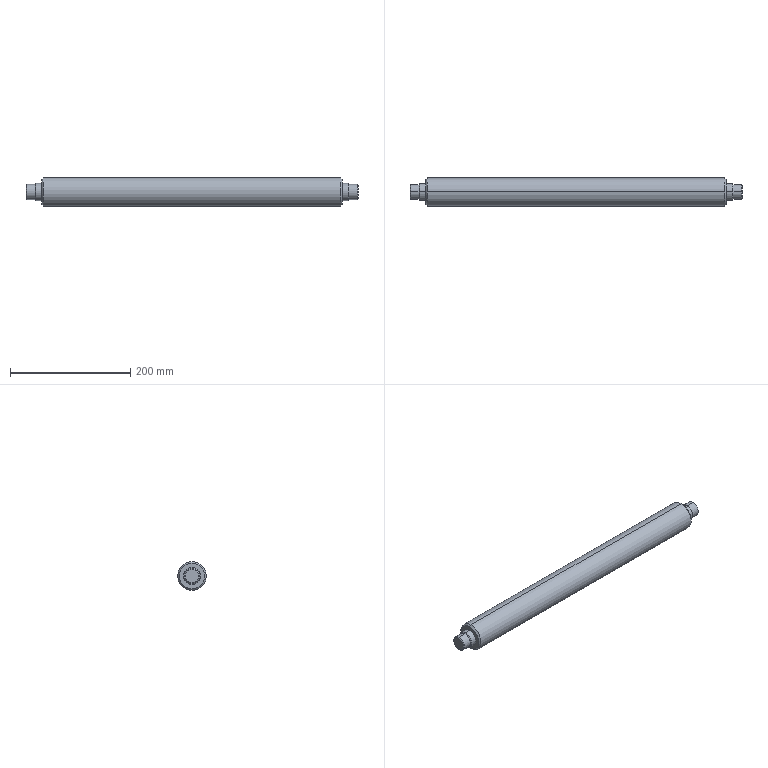Component | SolidWorks | DNR-71M20100BBEF2xx-A_509706-1 | 1 solid | 28 faces | box 552.45 x 47.63 x 47.63 mm | volume 918379 mm3 | cone 12 | cylinder 10 | plane 6 | commonest cylinder face diameters 25.019 x4 28.448 x4 47.625 x2
STEP:
#1=COLOUR_RGB('',0.7922,0.8196,0.9333);
#2=FILL_AREA_STYLE_COLOUR('',#1);
#3=FILL_AREA_STYLE('',(#2));
#4=SURFACE_STYLE_FILL_AREA(#3);
#5=SURFACE_SIDE_STYLE('',(#4));
#6=SURFACE_STYLE_USAGE(.BOTH.,#5);
#7=PRESENTATION_STYLE_ASSIGNMENT((#6));
#8=CARTESIAN_POINT('',(10.285,-5.162,4.758));
#9=VERTEX_POINT('',#8);
#10=CARTESIAN_POINT('',(10.285,-5.162,5.778));
#11=VERTEX_POINT('',#10);
#12=CARTESIAN_POINT('',(10.285,-5.162,5.268));
#13=DIRECTION('',(1.,0.,0.));
#14=DIRECTION('',(0.,0.,-1.));
#15=AXIS2_PLACEMENT_3D('',#12,#13,#14);
#16=CIRCLE('',#15,0.51);
#17=EDGE_CURVE('',#9,#11,#16,.T.);
#18=ORIENTED_EDGE('',*,*,#17,.F.);
#19=CARTESIAN_POINT('',(10.235,-5.162,4.708));
#20=VERTEX_POINT('',#19);
#21=CARTESIAN_POINT('',(10.285,-5.162,4.758));
#22=DIRECTION('',(-0.7071,0.,-0.7071));
#23=VECTOR('',#22,39.37);
#24=LINE('',#21,#23);
#25=EDGE_CURVE('',#9,#20,#24,.T.);
#26=ORIENTED_EDGE('',*,*,#25,.T.);
#27=CARTESIAN_POINT('',(10.235,-5.162,5.828));
#28=VERTEX_POINT('',#27);
#29=CARTESIAN_POINT('',(10.235,-5.162,5.268));
#30=DIRECTION('',(-1.,0.,0.));
#31=DIRECTION('',(0.,0.,-1.));
#32=AXIS2_PLACEMENT_3D('',#29,#30,#31);
#33=CIRCLE('',#32,0.56);
#34=EDGE_CURVE('',#28,#20,#33,.T.);
#35=ORIENTED_EDGE('',*,*,#34,.F.);
#36=CARTESIAN_POINT('',(10.285,-5.162,5.778));
#37=DIRECTION('',(-0.7071,0.,0.7071));
#38=VECTOR('',#37,39.37);
#39=LINE('',#36,#38);
#40=EDGE_CURVE('',#11,#28,#39,.T.);
#41=ORIENTED_EDGE('',*,*,#40,.F.);
#42=EDGE_LOOP('',(#18,#26,#35,#41));
#43=FACE_OUTER_BOUND('',#42,.T.);
#44=CARTESIAN_POINT('',(10.285,-5.162,5.268));
#45=DIRECTION('',(-1.,0.,0.));
#46=DIRECTION('',(0.,0.,1.));
#47=AXIS2_PLACEMENT_3D('',#44,#45,#46);
#48=CONICAL_SURFACE('',#47,0.51,0.7854);
#49=ADVANCED_FACE('',(#43),#48,.T.);
#50=CARTESIAN_POINT('',(-10.285,-5.162,5.778));
#51=VERTEX_POINT('',#50);
#52=CARTESIAN_POINT('',(-10.285,-5.162,4.758));
#53=VERTEX_POINT('',#52);
#54=CARTESIAN_POINT('',(-10.285,-5.162,5.268));
#55=DIRECTION('',(-1.,0.,0.));
#56=DIRECTION('',(0.,0.,1.));
#57=AXIS2_PLACEMENT_3D('',#54,#55,#56);
#58=CIRCLE('',#57,0.51);
#59=EDGE_CURVE('',#51,#53,#58,.T.);
#60=ORIENTED_EDGE('',*,*,#59,.F.);
#61=CARTESIAN_POINT('',(-10.235,-5.162,5.828));
#62=VERTEX_POINT('',#61);
#63=CARTESIAN_POINT('',(-10.235,-5.162,5.828));
#64=DIRECTION('',(0.7071,0.,0.7071));
#65=VECTOR('',#64,39.37);
#66=LINE('',#63,#65);
#67=EDGE_CURVE('',#51,#62,#66,.T.);
#68=ORIENTED_EDGE('',*,*,#67,.T.);
#69=CARTESIAN_POINT('',(-10.235,-5.162,4.708));
#70=VERTEX_POINT('',#69);
#71=CARTESIAN_POINT('',(-10.235,-5.162,5.268));
#72=DIRECTION('',(1.,0.,0.));
#73=DIRECTION('',(0.,0.,1.));
#74=AXIS2_PLACEMENT_3D('',#71,#72,#73);
#75=CIRCLE('',#74,0.56);
#76=EDGE_CURVE('',#70,#62,#75,.T.);
#77=ORIENTED_EDGE('',*,*,#76,.F.);
#78=CARTESIAN_POINT('',(-10.235,-5.162,4.708));
#79=DIRECTION('',(0.7071,0.,-0.7071));
#80=VECTOR('',#79,39.37);
#81=LINE('',#78,#80);
#82=EDGE_CURVE('',#53,#70,#81,.T.);
#83=ORIENTED_EDGE('',*,*,#82,.F.);
#84=EDGE_LOOP('',(#60,#68,#77,#83));
#85=FACE_OUTER_BOUND('',#84,.T.);
#86=CARTESIAN_POINT('',(-10.235,-5.162,5.268));
#87=DIRECTION('',(1.,0.,0.));
#88=DIRECTION('',(0.,0.,-1.));
#89=AXIS2_PLACEMENT_3D('',#86,#87,#88);
#90=CONICAL_SURFACE('',#89,0.56,0.7854);
#91=ADVANCED_FACE('',(#85),#90,.T.);
#92=CARTESIAN_POINT('',(10.875,-5.162,4.825));
#93=VERTEX_POINT('',#92);
#94=CARTESIAN_POINT('',(10.875,-5.162,5.71));
#95=VERTEX_POINT('',#94);
#96=CARTESIAN_POINT('',(10.875,-5.162,5.268));
#97=DIRECTION('',(1.,0.,0.));
#98=DIRECTION('',(0.,0.,-1.));
#99=AXIS2_PLACEMENT_3D('',#96,#97,#98);
#100=CIRCLE('',#99,0.4425);
#101=EDGE_CURVE('',#93,#95,#100,.T.);
#102=ORIENTED_EDGE('',*,*,#101,.F.);
#103=CARTESIAN_POINT('',(10.825,-5.162,4.775));
#104=VERTEX_POINT('',#103);
#105=CARTESIAN_POINT('',(10.875,-5.162,4.825));
#106=DIRECTION('',(-0.7071,0.,-0.7071));
#107=VECTOR('',#106,39.37);
#108=LINE('',#105,#107);
#109=EDGE_CURVE('',#93,#104,#108,.T.);
#110=ORIENTED_EDGE('',*,*,#109,.T.);
#111=CARTESIAN_POINT('',(10.825,-5.162,5.76));
#112=VERTEX_POINT('',#111);
#113=CARTESIAN_POINT('',(10.825,-5.162,5.268));
#114=DIRECTION('',(-1.,0.,0.));
#115=DIRECTION('',(0.,0.,-1.));
#116=AXIS2_PLACEMENT_3D('',#113,#114,#115);
#117=CIRCLE('',#116,0.4925);
#118=EDGE_CURVE('',#112,#104,#117,.T.);
#119=ORIENTED_EDGE('',*,*,#118,.F.);
#120=CARTESIAN_POINT('',(10.875,-5.162,5.71));
#121=DIRECTION('',(-0.7071,0.,0.7071));
#122=VECTOR('',#121,39.37);
#123=LINE('',#120,#122);
#124=EDGE_CURVE('',#95,#112,#123,.T.);
#125=ORIENTED_EDGE('',*,*,#124,.F.);
#126=EDGE_LOOP('',(#102,#110,#119,#125));
#127=FACE_OUTER_BOUND('',#126,.T.);
#128=CARTESIAN_POINT('',(10.875,-5.162,5.268));
#129=DIRECTION('',(-1.,0.,0.));
#130=DIRECTION('',(0.,0.,1.));
#131=AXIS2_PLACEMENT_3D('',#128,#129,#130);
#132=CONICAL_SURFACE('',#131,0.4425,0.7854);
#133=ADVANCED_FACE('',(#127),#132,.T.);
#134=CARTESIAN_POINT('',(-10.875,-5.162,5.71));
#135=VERTEX_POINT('',#134);
#136=CARTESIAN_POINT('',(-10.875,-5.162,4.825));
#137=VERTEX_POINT('',#136);
#138=CARTESIAN_POINT('',(-10.875,-5.162,5.268));
#139=DIRECTION('',(-1.,0.,0.));
#140=DIRECTION('',(0.,0.,1.));
#141=AXIS2_PLACEMENT_3D('',#138,#139,#140);
#142=CIRCLE('',#141,0.4425);
#143=EDGE_CURVE('',#135,#137,#142,.T.);
#144=ORIENTED_EDGE('',*,*,#143,.F.);
#145=CARTESIAN_POINT('',(-10.825,-5.162,5.76));
#146=VERTEX_POINT('',#145);
#147=CARTESIAN_POINT('',(-10.825,-5.162,5.76));
#148=DIRECTION('',(0.7071,0.,0.7071));
#149=VECTOR('',#148,39.37);
#150=LINE('',#147,#149);
#151=EDGE_CURVE('',#135,#146,#150,.T.);
#152=ORIENTED_EDGE('',*,*,#151,.T.);
#153=CARTESIAN_POINT('',(-10.825,-5.162,4.775));
#154=VERTEX_POINT('',#153);
#155=CARTESIAN_POINT('',(-10.825,-5.162,5.268));
#156=DIRECTION('',(1.,0.,0.));
#157=DIRECTION('',(0.,0.,1.));
#158=AXIS2_PLACEMENT_3D('',#155,#156,#157);
#159=CIRCLE('',#158,0.4925);
#160=EDGE_CURVE('',#154,#146,#159,.T.);
#161=ORIENTED_EDGE('',*,*,#160,.F.);
#162=CARTESIAN_POINT('',(-10.825,-5.162,4.775));
#163=DIRECTION('',(0.7071,0.,-0.7071));
#164=VECTOR('',#163,39.37);
#165=LINE('',#162,#164);
#166=EDGE_CURVE('',#137,#154,#165,.T.);
#167=ORIENTED_EDGE('',*,*,#166,.F.);
#168=EDGE_LOOP('',(#144,#152,#161,#167));
#169=FACE_OUTER_BOUND('',#168,.T.);
#170=CARTESIAN_POINT('',(-10.825,-5.162,5.268));
#171=DIRECTION('',(1.,0.,0.));
#172=DIRECTION('',(0.,0.,-1.));
#173=AXIS2_PLACEMENT_3D('',#170,#171,#172);
#174=CONICAL_SURFACE('',#173,0.4925,0.7854);
#175=ADVANCED_FACE('',(#169),#174,.T.);
#176=CARTESIAN_POINT('',(9.84,-5.162,4.43));
#177=VERTEX_POINT('',#176);
#178=CARTESIAN_POINT('',(9.84,-5.162,6.105));
#179=VERTEX_POINT('',#178);
#180=CARTESIAN_POINT('',(9.84,-5.162,5.268));
#181=DIRECTION('',(1.,0.,0.));
#182=DIRECTION('',(0.,0.,-1.));
#183=AXIS2_PLACEMENT_3D('',#180,#181,#182);
#184=CIRCLE('',#183,0.8375);
#185=EDGE_CURVE('',#177,#179,#184,.T.);
#186=ORIENTED_EDGE('',*,*,#185,.F.);
#187=CARTESIAN_POINT('',(9.74,-5.162,4.33));
#188=VERTEX_POINT('',#187);
#189=CARTESIAN_POINT('',(9.84,-5.162,4.43));
#190=DIRECTION('',(-0.7071,0.,-0.7071));
#191=VECTOR('',#190,39.37);
#192=LINE('',#189,#191);
#193=EDGE_CURVE('',#177,#188,#192,.T.);
#194=ORIENTED_EDGE('',*,*,#193,.T.);
#195=CARTESIAN_POINT('',(9.74,-5.162,6.205));
#196=VERTEX_POINT('',#195);
#197=CARTESIAN_POINT('',(9.74,-5.162,5.268));
#198=DIRECTION('',(-1.,0.,0.));
#199=DIRECTION('',(0.,0.,-1.));
#200=AXIS2_PLACEMENT_3D('',#197,#198,#199);
#201=CIRCLE('',#200,0.9375);
#202=EDGE_CURVE('',#196,#188,#201,.T.);
#203=ORIENTED_EDGE('',*,*,#202,.F.);
#204=CARTESIAN_POINT('',(9.84,-5.162,6.105));
#205=DIRECTION('',(-0.7071,0.,0.7071));
#206=VECTOR('',#205,39.37);
#207=LINE('',#204,#206);
#208=EDGE_CURVE('',#179,#196,#207,.T.);
#209=ORIENTED_EDGE('',*,*,#208,.F.);
#210=EDGE_LOOP('',(#186,#194,#203,#209));
#211=FACE_OUTER_BOUND('',#210,.T.);
#212=CARTESIAN_POINT('',(9.84,-5.162,5.268));
#213=DIRECTION('',(-1.,0.,0.));
#214=DIRECTION('',(0.,0.,1.));
#215=AXIS2_PLACEMENT_3D('',#212,#213,#214);
#216=CONICAL_SURFACE('',#215,0.8375,0.7854);
#217=ADVANCED_FACE('',(#211),#216,.T.);
#218=CARTESIAN_POINT('',(-9.84,-5.162,6.105));
#219=VERTEX_POINT('',#218);
#220=CARTESIAN_POINT('',(-9.84,-5.162,4.43));
#221=VERTEX_POINT('',#220);
#222=CARTESIAN_POINT('',(-9.84,-5.162,5.268));
#223=DIRECTION('',(-1.,0.,0.));
#224=DIRECTION('',(0.,0.,1.));
#225=AXIS2_PLACEMENT_3D('',#222,#223,#224);
#226=CIRCLE('',#225,0.8375);
#227=EDGE_CURVE('',#219,#221,#226,.T.);
#228=ORIENTED_EDGE('',*,*,#227,.F.);
#229=CARTESIAN_POINT('',(-9.74,-5.162,6.205));
#230=VERTEX_POINT('',#229);
#231=CARTESIAN_POINT('',(-9.74,-5.162,6.205));
#232=DIRECTION('',(0.7071,0.,0.7071));
#233=VECTOR('',#232,39.37);
#234=LINE('',#231,#233);
#235=EDGE_CURVE('',#219,#230,#234,.T.);
#236=ORIENTED_EDGE('',*,*,#235,.T.);
#237=CARTESIAN_POINT('',(-9.74,-5.162,4.33));
#238=VERTEX_POINT('',#237);
#239=CARTESIAN_POINT('',(-9.74,-5.162,5.268));
#240=DIRECTION('',(1.,0.,0.));
#241=DIRECTION('',(0.,0.,1.));
#242=AXIS2_PLACEMENT_3D('',#239,#240,#241);
#243=CIRCLE('',#242,0.9375);
#244=EDGE_CURVE('',#238,#230,#243,.T.);
#245=ORIENTED_EDGE('',*,*,#244,.F.);
#246=CARTESIAN_POINT('',(-9.74,-5.162,4.33));
#247=DIRECTION('',(0.7071,0.,-0.7071));
#248=VECTOR('',#247,39.37);
#249=LINE('',#246,#248);
#250=EDGE_CURVE('',#221,#238,#249,.T.);
#251=ORIENTED_EDGE('',*,*,#250,.F.);
#252=EDGE_LOOP('',(#228,#236,#245,#251));
#253=FACE_OUTER_BOUND('',#252,.T.);
#254=CARTESIAN_POINT('',(-9.74,-5.162,5.268));
#255=DIRECTION('',(1.,0.,0.));
#256=DIRECTION('',(0.,0.,-1.));
#257=AXIS2_PLACEMENT_3D('',#254,#255,#256);
#258=CONICAL_SURFACE('',#257,0.9375,0.7854);
#259=ADVANCED_FACE('',(#253),#258,.T.);
#260=CARTESIAN_POINT('',(10.285,-5.162,4.775));
#261=VERTEX_POINT('',#260);
#262=CARTESIAN_POINT('',(10.285,-5.162,5.76));
#263=VERTEX_POINT('',#262);
#264=CARTESIAN_POINT('',(10.285,-5.162,5.268));
#265=DIRECTION('',(1.,0.,0.));
#266=DIRECTION('',(0.,0.,-1.));
#267=AXIS2_PLACEMENT_3D('',#264,#265,#266);
#268=CIRCLE('',#267,0.4925);
#269=EDGE_CURVE('',#261,#263,#268,.T.);
#270=ORIENTED_EDGE('',*,*,#269,.T.);
#271=CARTESIAN_POINT('',(10.875,-5.162,5.76));
#272=DIRECTION('',(1.,0.,0.));
#273=VECTOR('',#272,39.37);
#274=LINE('',#271,#273);
#275=EDGE_CURVE('',#263,#112,#274,.T.);
#276=ORIENTED_EDGE('',*,*,#275,.T.);
#277=ORIENTED_EDGE('',*,*,#118,.T.);
#278=CARTESIAN_POINT('',(10.875,-5.162,4.775));
#279=DIRECTION('',(1.,0.,0.));
#280=VECTOR('',#279,39.37);
#281=LINE('',#278,#280);
#282=EDGE_CURVE('',#261,#104,#281,.T.);
#283=ORIENTED_EDGE('',*,*,#282,.F.);
#284=EDGE_LOOP('',(#270,#276,#277,#283));
#285=FACE_OUTER_BOUND('',#284,.T.);
#286=CARTESIAN_POINT('',(10.875,-5.162,5.268));
#287=DIRECTION('',(1.,0.,0.));
#288=DIRECTION('',(0.,0.,-1.));
#289=AXIS2_PLACEMENT_3D('',#286,#287,#288);
#290=CYLINDRICAL_SURFACE('',#289,0.4925);
#291=ADVANCED_FACE('',(#285),#290,.T.);
#292=CARTESIAN_POINT('',(9.84,-5.162,4.708));
#293=VERTEX_POINT('',#292);
#294=CARTESIAN_POINT('',(9.84,-5.162,5.828));
#295=VERTEX_POINT('',#294);
#296=CARTESIAN_POINT('',(9.84,-5.162,5.268));
#297=DIRECTION('',(1.,0.,0.));
#298=DIRECTION('',(0.,0.,-1.));
#299=AXIS2_PLACEMENT_3D('',#296,#297,#298);
#300=CIRCLE('',#299,0.56);
#301=EDGE_CURVE('',#293,#295,#300,.T.);
#302=ORIENTED_EDGE('',*,*,#301,.T.);
#303=CARTESIAN_POINT('',(10.875,-5.162,5.828));
#304=DIRECTION('',(1.,0.,0.));
#305=VECTOR('',#304,39.37);
#306=LINE('',#303,#305);
#307=EDGE_CURVE('',#295,#28,#306,.T.);
#308=ORIENTED_EDGE('',*,*,#307,.T.);
#309=ORIENTED_EDGE('',*,*,#34,.T.);
#310=CARTESIAN_POINT('',(10.875,-5.162,4.708));
#311=DIRECTION('',(1.,0.,0.));
#312=VECTOR('',#311,39.37);
#313=LINE('',#310,#312);
#314=EDGE_CURVE('',#293,#20,#313,.T.);
#315=ORIENTED_EDGE('',*,*,#314,.F.);
#316=EDGE_LOOP('',(#302,#308,#309,#315));
#317=FACE_OUTER_BOUND('',#316,.T.);
#318=CARTESIAN_POINT('',(10.875,-5.162,5.268));
#319=DIRECTION('',(1.,0.,0.));
#320=DIRECTION('',(0.,0.,-1.));
#321=AXIS2_PLACEMENT_3D('',#318,#319,#320);
#322=CYLINDRICAL_SURFACE('',#321,0.56);
#323=ADVANCED_FACE('',(#317),#322,.T.);
#324=ORIENTED_EDGE('',*,*,#244,.T.);
#325=CARTESIAN_POINT('',(10.875,-5.162,6.205));
#326=DIRECTION('',(1.,0.,0.));
#327=VECTOR('',#326,39.37);
#328=LINE('',#325,#327);
#329=EDGE_CURVE('',#230,#196,#328,.T.);
#330=ORIENTED_EDGE('',*,*,#329,.T.);
#331=ORIENTED_EDGE('',*,*,#202,.T.);
#332=CARTESIAN_POINT('',(10.875,-5.162,4.33));
#333=DIRECTION('',(1.,0.,0.));
#334=VECTOR('',#333,39.37);
#335=LINE('',#332,#334);
#336=EDGE_CURVE('',#238,#188,#335,.T.);
#337=ORIENTED_EDGE('',*,*,#336,.F.);
#338=EDGE_LOOP('',(#324,#330,#331,#337));
#339=FACE_OUTER_BOUND('',#338,.T.);
#340=CARTESIAN_POINT('',(10.875,-5.162,5.268));
#341=DIRECTION('',(1.,0.,0.));
#342=DIRECTION('',(0.,0.,-1.));
#343=AXIS2_PLACEMENT_3D('',#340,#341,#342);
#344=CYLINDRICAL_SURFACE('',#343,0.9375);
#345=ADVANCED_FACE('',(#339),#344,.T.);
#346=ORIENTED_EDGE('',*,*,#76,.T.);
#347=CARTESIAN_POINT('',(-9.84,-5.162,5.828));
#348=VERTEX_POINT('',#347);
#349=CARTESIAN_POINT('',(10.875,-5.162,5.828));
#350=DIRECTION('',(1.,0.,0.));
#351=VECTOR('',#350,39.37);
#352=LINE('',#349,#351);
#353=EDGE_CURVE('',#62,#348,#352,.T.);
#354=ORIENTED_EDGE('',*,*,#353,.T.);
#355=CARTESIAN_POINT('',(-9.84,-5.162,4.708));
#356=VERTEX_POINT('',#355);
#357=CARTESIAN_POINT('',(-9.84,-5.162,5.268));
#358=DIRECTION('',(1.,0.,0.));
#359=DIRECTION('',(0.,0.,-1.));
#360=AXIS2_PLACEMENT_3D('',#357,#358,#359);
#361=CIRCLE('',#360,0.56);
#362=EDGE_CURVE('',#356,#348,#361,.T.);
#363=ORIENTED_EDGE('',*,*,#362,.F.);
#364=CARTESIAN_POINT('',(10.875,-5.162,4.708));
#365=DIRECTION('',(1.,0.,0.));
#366=VECTOR('',#365,39.37);
#367=LINE('',#364,#366);
#368=EDGE_CURVE('',#70,#356,#367,.T.);
#369=ORIENTED_EDGE('',*,*,#368,.F.);
#370=EDGE_LOOP('',(#346,#354,#363,#369));
#371=FACE_OUTER_BOUND('',#370,.T.);
#372=CARTESIAN_POINT('',(10.875,-5.162,5.268));
#373=DIRECTION('',(1.,0.,0.));
#374=DIRECTION('',(0.,0.,-1.));
#375=AXIS2_PLACEMENT_3D('',#372,#373,#374);
#376=CYLINDRICAL_SURFACE('',#375,0.56);
#377=ADVANCED_FACE('',(#371),#376,.T.);
#378=ORIENTED_EDGE('',*,*,#160,.T.);
#379=CARTESIAN_POINT('',(-10.285,-5.162,5.76));
#380=VERTEX_POINT('',#379);
#381=CARTESIAN_POINT('',(10.875,-5.162,5.76));
#382=DIRECTION('',(1.,0.,0.));
#383=VECTOR('',#382,39.37);
#384=LINE('',#381,#383);
#385=EDGE_CURVE('',#146,#380,#384,.T.);
#386=ORIENTED_EDGE('',*,*,#385,.T.);
#387=CARTESIAN_POINT('',(-10.285,-5.162,4.775));
#388=VERTEX_POINT('',#387);
#389=CARTESIAN_POINT('',(-10.285,-5.162,5.268));
#390=DIRECTION('',(1.,0.,0.));
#391=DIRECTION('',(0.,0.,-1.));
#392=AXIS2_PLACEMENT_3D('',#389,#390,#391);
#393=CIRCLE('',#392,0.4925);
#394=EDGE_CURVE('',#388,#380,#393,.T.);
#395=ORIENTED_EDGE('',*,*,#394,.F.);
#396=CARTESIAN_POINT('',(10.875,-5.162,4.775));
#397=DIRECTION('',(1.,0.,0.));
#398=VECTOR('',#397,39.37);
#399=LINE('',#396,#398);
#400=EDGE_CURVE('',#154,#388,#399,.T.);
#401=ORIENTED_EDGE('',*,*,#400,.F.);
#402=EDGE_LOOP('',(#378,#386,#395,#401));
#403=FACE_OUTER_BOUND('',#402,.T.);
#404=CARTESIAN_POINT('',(10.875,-5.162,5.268));
#405=DIRECTION('',(1.,0.,0.));
#406=DIRECTION('',(0.,0.,-1.));
#407=AXIS2_PLACEMENT_3D('',#404,#405,#406);
#408=CYLINDRICAL_SURFACE('',#407,0.4925);
#409=ADVANCED_FACE('',(#403),#408,.T.);
#410=CARTESIAN_POINT('',(-10.875,-5.162,5.268));
#411=DIRECTION('',(-1.,0.,0.));
#412=DIRECTION('',(0.,0.,1.));
#413=AXIS2_PLACEMENT_3D('',#410,#411,#412);
#414=CIRCLE('',#413,0.4425);
#415=EDGE_CURVE('',#137,#135,#414,.T.);
#416=ORIENTED_EDGE('',*,*,#415,.T.);
#417=ORIENTED_EDGE('',*,*,#143,.T.);
#418=EDGE_LOOP('',(#416,#417));
#419=FACE_OUTER_BOUND('',#418,.T.);
#420=CARTESIAN_POINT('',(-10.875,-4.67,5.268));
#421=DIRECTION('',(-1.,0.,0.));
#422=DIRECTION('',(0.,0.,1.));
#423=AXIS2_PLACEMENT_3D('',#420,#421,#422);
#424=PLANE('',#423);
#425=ADVANCED_FACE('',(#419),#424,.T.);
#426=ORIENTED_EDGE('',*,*,#385,.F.);
#427=CARTESIAN_POINT('',(-10.825,-5.162,5.268));
#428=DIRECTION('',(1.,0.,0.));
#429=DIRECTION('',(0.,0.,1.));
#430=AXIS2_PLACEMENT_3D('',#427,#428,#429);
#431=CIRCLE('',#430,0.4925);
#432=EDGE_CURVE('',#146,#154,#431,.T.);
#433=ORIENTED_EDGE('',*,*,#432,.T.);
#434=ORIENTED_EDGE('',*,*,#400,.T.);
#435=CARTESIAN_POINT('',(-10.285,-5.162,5.268));
#436=DIRECTION('',(1.,0.,0.));
#437=DIRECTION('',(0.,0.,-1.));
#438=AXIS2_PLACEMENT_3D('',#435,#436,#437);
#439=CIRCLE('',#438,0.4925);
#440=EDGE_CURVE('',#380,#388,#439,.T.);
#441=ORIENTED_EDGE('',*,*,#440,.F.);
#442=EDGE_LOOP('',(#426,#433,#434,#441));
#443=FACE_OUTER_BOUND('',#442,.T.);
#444=CARTESIAN_POINT('',(10.875,-5.162,5.268));
#445=DIRECTION('',(1.,0.,0.));
#446=DIRECTION('',(0.,0.,-1.));
#447=AXIS2_PLACEMENT_3D('',#444,#445,#446);
#448=CYLINDRICAL_SURFACE('',#447,0.4925);
#449=ADVANCED_FACE('',(#443),#448,.T.);
#450=CARTESIAN_POINT('',(-10.285,-5.162,5.268));
#451=DIRECTION('',(-1.,0.,0.));
#452=DIRECTION('',(0.,0.,1.));
#453=AXIS2_PLACEMENT_3D('',#450,#451,#452);
#454=CIRCLE('',#453,0.51);
#455=EDGE_CURVE('',#53,#51,#454,.T.);
#456=ORIENTED_EDGE('',*,*,#455,.T.);
#457=ORIENTED_EDGE('',*,*,#59,.T.);
#458=EDGE_LOOP('',(#456,#457));
#459=FACE_OUTER_BOUND('',#458,.T.);
#460=ORIENTED_EDGE('',*,*,#394,.T.);
#461=ORIENTED_EDGE('',*,*,#440,.T.);
#462=EDGE_LOOP('',(#460,#461));
#463=FACE_BOUND('',#462,.T.);
#464=CARTESIAN_POINT('',(-10.285,-4.67,5.268));
#465=DIRECTION('',(-1.,0.,0.));
#466=DIRECTION('',(0.,0.,1.));
#467=AXIS2_PLACEMENT_3D('',#464,#465,#466);
#468=PLANE('',#467);
#469=ADVANCED_FACE('',(#459,#463),#468,.T.);
#470=ORIENTED_EDGE('',*,*,#353,.F.);
#471=CARTESIAN_POINT('',(-10.235,-5.162,5.268));
#472=DIRECTION('',(1.,0.,0.));
#473=DIRECTION('',(0.,0.,1.));
#474=AXIS2_PLACEMENT_3D('',#471,#472,#473);
#475=CIRCLE('',#474,0.56);
#476=EDGE_CURVE('',#62,#70,#475,.T.);
#477=ORIENTED_EDGE('',*,*,#476,.T.);
#478=ORIENTED_EDGE('',*,*,#368,.T.);
#479=CARTESIAN_POINT('',(-9.84,-5.162,5.268));
#480=DIRECTION('',(1.,0.,0.));
#481=DIRECTION('',(0.,0.,-1.));
#482=AXIS2_PLACEMENT_3D('',#479,#480,#481);
#483=CIRCLE('',#482,0.56);
#484=EDGE_CURVE('',#348,#356,#483,.T.);
#485=ORIENTED_EDGE('',*,*,#484,.F.);
#486=EDGE_LOOP('',(#470,#477,#478,#485));
#487=FACE_OUTER_BOUND('',#486,.T.);
#488=CARTESIAN_POINT('',(10.875,-5.162,5.268));
#489=DIRECTION('',(1.,0.,0.));
#490=DIRECTION('',(0.,0.,-1.));
#491=AXIS2_PLACEMENT_3D('',#488,#489,#490);
#492=CYLINDRICAL_SURFACE('',#491,0.56);
#493=ADVANCED_FACE('',(#487),#492,.T.);
#494=CARTESIAN_POINT('',(-9.84,-5.162,5.268));
#495=DIRECTION('',(-1.,0.,0.));
#496=DIRECTION('',(0.,0.,1.));
#497=AXIS2_PLACEMENT_3D('',#494,#495,#496);
#498=CIRCLE('',#497,0.8375);
#499=EDGE_CURVE('',#221,#219,#498,.T.);
#500=ORIENTED_EDGE('',*,*,#499,.T.);
#501=ORIENTED_EDGE('',*,*,#227,.T.);
#502=EDGE_LOOP('',(#500,#501));
#503=FACE_OUTER_BOUND('',#502,.T.);
#504=ORIENTED_EDGE('',*,*,#362,.T.);
#505=ORIENTED_EDGE('',*,*,#484,.T.);
#506=EDGE_LOOP('',(#504,#505));
#507=FACE_BOUND('',#506,.T.);
#508=CARTESIAN_POINT('',(-9.84,-4.602,5.268));
#509=DIRECTION('',(-1.,0.,0.));
#510=DIRECTION('',(0.,0.,1.));
#511=AXIS2_PLACEMENT_3D('',#508,#509,#510);
#512=PLANE('',#511);
#513=ADVANCED_FACE('',(#503,#507),#512,.T.);
#514=ORIENTED_EDGE('',*,*,#329,.F.);
#515=CARTESIAN_POINT('',(-9.74,-5.162,5.268));
#516=DIRECTION('',(1.,0.,0.));
#517=DIRECTION('',(0.,0.,1.));
#518=AXIS2_PLACEMENT_3D('',#515,#516,#517);
#519=CIRCLE('',#518,0.9375);
#520=EDGE_CURVE('',#230,#238,#519,.T.);
#521=ORIENTED_EDGE('',*,*,#520,.T.);
#522=ORIENTED_EDGE('',*,*,#336,.T.);
#523=CARTESIAN_POINT('',(9.74,-5.162,5.268));
#524=DIRECTION('',(-1.,0.,0.));
#525=DIRECTION('',(0.,0.,-1.));
#526=AXIS2_PLACEMENT_3D('',#523,#524,#525);
#527=CIRCLE('',#526,0.9375);
#528=EDGE_CURVE('',#188,#196,#527,.T.);
#529=ORIENTED_EDGE('',*,*,#528,.T.);
#530=EDGE_LOOP('',(#514,#521,#522,#529));
#531=FACE_OUTER_BOUND('',#530,.T.);
#532=CARTESIAN_POINT('',(10.875,-5.162,5.268));
#533=DIRECTION('',(1.,0.,0.));
#534=DIRECTION('',(0.,0.,-1.));
#535=AXIS2_PLACEMENT_3D('',#532,#533,#534);
#536=CYLINDRICAL_SURFACE('',#535,0.9375);
#537=ADVANCED_FACE('',(#531),#536,.T.);
#538=CARTESIAN_POINT('',(9.84,-5.162,5.268));
#539=DIRECTION('',(1.,0.,0.));
#540=DIRECTION('',(0.,0.,-1.));
#541=AXIS2_PLACEMENT_3D('',#538,#539,#540);
#542=CIRCLE('',#541,0.8375);
#543=EDGE_CURVE('',#179,#177,#542,.T.);
#544=ORIENTED_EDGE('',*,*,#543,.T.);
#545=ORIENTED_EDGE('',*,*,#185,.T.);
#546=EDGE_LOOP('',(#544,#545));
#547=FACE_OUTER_BOUND('',#546,.T.);
#548=ORIENTED_EDGE('',*,*,#301,.F.);
#549=CARTESIAN_POINT('',(9.84,-5.162,5.268));
#550=DIRECTION('',(1.,0.,0.));
#551=DIRECTION('',(0.,0.,-1.));
#552=AXIS2_PLACEMENT_3D('',#549,#550,#551);
#553=CIRCLE('',#552,0.56);
#554=EDGE_CURVE('',#295,#293,#553,.T.);
#555=ORIENTED_EDGE('',*,*,#554,.F.);
#556=EDGE_LOOP('',(#548,#555));
#557=FACE_BOUND('',#556,.T.);
#558=CARTESIAN_POINT('',(9.84,-4.602,5.268));
#559=DIRECTION('',(1.,0.,0.));
#560=DIRECTION('',(0.,0.,-1.));
#561=AXIS2_PLACEMENT_3D('',#558,#559,#560);
#562=PLANE('',#561);
#563=ADVANCED_FACE('',(#547,#557),#562,.T.);
#564=ORIENTED_EDGE('',*,*,#307,.F.);
#565=ORIENTED_EDGE('',*,*,#554,.T.);
#566=ORIENTED_EDGE('',*,*,#314,.T.);
#567=CARTESIAN_POINT('',(10.235,-5.162,5.268));
#568=DIRECTION('',(-1.,0.,0.));
#569=DIRECTION('',(0.,0.,-1.));
#570=AXIS2_PLACEMENT_3D('',#567,#568,#569);
#571=CIRCLE('',#570,0.56);
#572=EDGE_CURVE('',#20,#28,#571,.T.);
#573=ORIENTED_EDGE('',*,*,#572,.T.);
#574=EDGE_LOOP('',(#564,#565,#566,#573));
#575=FACE_OUTER_BOUND('',#574,.T.);
#576=CARTESIAN_POINT('',(10.875,-5.162,5.268));
#577=DIRECTION('',(1.,0.,0.));
#578=DIRECTION('',(0.,0.,-1.));
#579=AXIS2_PLACEMENT_3D('',#576,#577,#578);
#580=CYLINDRICAL_SURFACE('',#579,0.56);
#581=ADVANCED_FACE('',(#575),#580,.T.);
#582=CARTESIAN_POINT('',(10.285,-5.162,5.268));
#583=DIRECTION('',(1.,0.,0.));
#584=DIRECTION('',(0.,0.,-1.));
#585=AXIS2_PLACEMENT_3D('',#582,#583,#584);
#586=CIRCLE('',#585,0.51);
#587=EDGE_CURVE('',#11,#9,#586,.T.);
#588=ORIENTED_EDGE('',*,*,#587,.T.);
#589=ORIENTED_EDGE('',*,*,#17,.T.);
#590=EDGE_LOOP('',(#588,#589));
#591=FACE_OUTER_BOUND('',#590,.T.);
#592=ORIENTED_EDGE('',*,*,#269,.F.);
#593=CARTESIAN_POINT('',(10.285,-5.162,5.268));
#594=DIRECTION('',(1.,0.,0.));
#595=DIRECTION('',(0.,0.,-1.));
#596=AXIS2_PLACEMENT_3D('',#593,#594,#595);
#597=CIRCLE('',#596,0.4925);
#598=EDGE_CURVE('',#263,#261,#597,.T.);
#599=ORIENTED_EDGE('',*,*,#598,.F.);
#600=EDGE_LOOP('',(#592,#599));
#601=FACE_BOUND('',#600,.T.);
#602=CARTESIAN_POINT('',(10.285,-4.67,5.268));
#603=DIRECTION('',(1.,0.,0.));
#604=DIRECTION('',(0.,0.,-1.));
#605=AXIS2_PLACEMENT_3D('',#602,#603,#604);
#606=PLANE('',#605);
#607=ADVANCED_FACE('',(#591,#601),#606,.T.);
#608=ORIENTED_EDGE('',*,*,#275,.F.);
#609=ORIENTED_EDGE('',*,*,#598,.T.);
#610=ORIENTED_EDGE('',*,*,#282,.T.);
#611=CARTESIAN_POINT('',(10.825,-5.162,5.268));
#612=DIRECTION('',(-1.,0.,0.));
#613=DIRECTION('',(0.,0.,-1.));
#614=AXIS2_PLACEMENT_3D('',#611,#612,#613);
#615=CIRCLE('',#614,0.4925);
#616=EDGE_CURVE('',#104,#112,#615,.T.);
#617=ORIENTED_EDGE('',*,*,#616,.T.);
#618=EDGE_LOOP('',(#608,#609,#610,#617));
#619=FACE_OUTER_BOUND('',#618,.T.);
#620=CARTESIAN_POINT('',(10.875,-5.162,5.268));
#621=DIRECTION('',(1.,0.,0.));
#622=DIRECTION('',(0.,0.,-1.));
#623=AXIS2_PLACEMENT_3D('',#620,#621,#622);
#624=CYLINDRICAL_SURFACE('',#623,0.4925);
#625=ADVANCED_FACE('',(#619),#624,.T.);
#626=CARTESIAN_POINT('',(10.875,-5.162,5.268));
#627=DIRECTION('',(1.,0.,0.));
#628=DIRECTION('',(0.,0.,-1.));
#629=AXIS2_PLACEMENT_3D('',#626,#627,#628);
#630=CIRCLE('',#629,0.4425);
#631=EDGE_CURVE('',#95,#93,#630,.T.);
#632=ORIENTED_EDGE('',*,*,#631,.T.);
#633=ORIENTED_EDGE('',*,*,#101,.T.);
#634=EDGE_LOOP('',(#632,#633));
#635=FACE_OUTER_BOUND('',#634,.T.);
#636=CARTESIAN_POINT('',(10.875,-4.67,5.268));
#637=DIRECTION('',(1.,0.,0.));
#638=DIRECTION('',(0.,0.,-1.));
#639=AXIS2_PLACEMENT_3D('',#636,#637,#638);
#640=PLANE('',#639);
#641=ADVANCED_FACE('',(#635),#640,.T.);
#642=ORIENTED_EDGE('',*,*,#235,.F.);
#643=ORIENTED_EDGE('',*,*,#499,.F.);
#644=ORIENTED_EDGE('',*,*,#250,.T.);
#645=ORIENTED_EDGE('',*,*,#520,.F.);
#646=EDGE_LOOP('',(#642,#643,#644,#645));
#647=FACE_OUTER_BOUND('',#646,.T.);
#648=CARTESIAN_POINT('',(-9.74,-5.162,5.268));
#649=DIRECTION('',(1.,0.,0.));
#650=DIRECTION('',(0.,0.,-1.));
#651=AXIS2_PLACEMENT_3D('',#648,#649,#650);
#652=CONICAL_SURFACE('',#651,0.9375,0.7854);
#653=ADVANCED_FACE('',(#647),#652,.T.);
#654=ORIENTED_EDGE('',*,*,#193,.F.);
#655=ORIENTED_EDGE('',*,*,#543,.F.);
#656=ORIENTED_EDGE('',*,*,#208,.T.);
#657=ORIENTED_EDGE('',*,*,#528,.F.);
#658=EDGE_LOOP('',(#654,#655,#656,#657));
#659=FACE_OUTER_BOUND('',#658,.T.);
#660=CARTESIAN_POINT('',(9.84,-5.162,5.268));
#661=DIRECTION('',(-1.,0.,0.));
#662=DIRECTION('',(0.,0.,1.));
#663=AXIS2_PLACEMENT_3D('',#660,#661,#662);
#664=CONICAL_SURFACE('',#663,0.8375,0.7854);
#665=ADVANCED_FACE('',(#659),#664,.T.);
#666=ORIENTED_EDGE('',*,*,#151,.F.);
#667=ORIENTED_EDGE('',*,*,#415,.F.);
#668=ORIENTED_EDGE('',*,*,#166,.T.);
#669=ORIENTED_EDGE('',*,*,#432,.F.);
#670=EDGE_LOOP('',(#666,#667,#668,#669));
#671=FACE_OUTER_BOUND('',#670,.T.);
#672=CARTESIAN_POINT('',(-10.825,-5.162,5.268));
#673=DIRECTION('',(1.,0.,0.));
#674=DIRECTION('',(0.,0.,-1.));
#675=AXIS2_PLACEMENT_3D('',#672,#673,#674);
#676=CONICAL_SURFACE('',#675,0.4925,0.7854);
#677=ADVANCED_FACE('',(#671),#676,.T.);
#678=ORIENTED_EDGE('',*,*,#109,.F.);
#679=ORIENTED_EDGE('',*,*,#631,.F.);
#680=ORIENTED_EDGE('',*,*,#124,.T.);
#681=ORIENTED_EDGE('',*,*,#616,.F.);
#682=EDGE_LOOP('',(#678,#679,#680,#681));
#683=FACE_OUTER_BOUND('',#682,.T.);
#684=CARTESIAN_POINT('',(10.875,-5.162,5.268));
#685=DIRECTION('',(-1.,0.,0.));
#686=DIRECTION('',(0.,0.,1.));
#687=AXIS2_PLACEMENT_3D('',#684,#685,#686);
#688=CONICAL_SURFACE('',#687,0.4425,0.7854);
#689=ADVANCED_FACE('',(#683),#688,.T.);
#690=ORIENTED_EDGE('',*,*,#67,.F.);
#691=ORIENTED_EDGE('',*,*,#455,.F.);
#692=ORIENTED_EDGE('',*,*,#82,.T.);
#693=ORIENTED_EDGE('',*,*,#476,.F.);
#694=EDGE_LOOP('',(#690,#691,#692,#693));
#695=FACE_OUTER_BOUND('',#694,.T.);
#696=CARTESIAN_POINT('',(-10.235,-5.162,5.268));
#697=DIRECTION('',(1.,0.,0.));
#698=DIRECTION('',(0.,0.,-1.));
#699=AXIS2_PLACEMENT_3D('',#696,#697,#698);
#700=CONICAL_SURFACE('',#699,0.56,0.7854);
#701=ADVANCED_FACE('',(#695),#700,.T.);
#702=ORIENTED_EDGE('',*,*,#25,.F.);
#703=ORIENTED_EDGE('',*,*,#587,.F.);
#704=ORIENTED_EDGE('',*,*,#40,.T.);
#705=ORIENTED_EDGE('',*,*,#572,.F.);
#706=EDGE_LOOP('',(#702,#703,#704,#705));
#707=FACE_OUTER_BOUND('',#706,.T.);
#708=CARTESIAN_POINT('',(10.285,-5.162,5.268));
#709=DIRECTION('',(-1.,0.,0.));
#710=DIRECTION('',(0.,0.,1.));
#711=AXIS2_PLACEMENT_3D('',#708,#709,#710);
#712=CONICAL_SURFACE('',#711,0.51,0.7854);
#713=ADVANCED_FACE('',(#707),#712,.T.);
#714=CLOSED_SHELL('',(#49,#91,#133,#175,#217,#259,#291,#323,#345,#377,#409,#425,#449,#469,#493,#513,#537,#563,#581,#607,#625,#641,#653,#665,#677,#689,#701,#713));
#715=MANIFOLD_SOLID_BREP('',#714);
#716=STYLED_ITEM('',(#7),#715);
#717=PRESENTATION_LAYER_ASSIGNMENT('','',(#716));
#718=(LENGTH_UNIT()NAMED_UNIT(*)SI_UNIT($,.METRE.));
#719=LENGTH_MEASURE_WITH_UNIT(LENGTH_MEASURE(0.0254),#718);
#720=DIMENSIONAL_EXPONENTS(1.,0.,0.,0.,0.,0.,0.);
#721=(CONVERSION_BASED_UNIT('',#719)LENGTH_UNIT()NAMED_UNIT(#720));
#722=UNCERTAINTY_MEASURE_WITH_UNIT(LENGTH_MEASURE(0.00001),#721,'','');
#723=(NAMED_UNIT(*)PLANE_ANGLE_UNIT()SI_UNIT($,.RADIAN.));
#724=(NAMED_UNIT(*)SI_UNIT($,.STERADIAN.)SOLID_ANGLE_UNIT());
#725=(GEOMETRIC_REPRESENTATION_CONTEXT(3)GLOBAL_UNCERTAINTY_ASSIGNED_CONTEXT((#722))GLOBAL_UNIT_ASSIGNED_CONTEXT((#721,#723,#724))REPRESENTATION_CONTEXT('',''));
#726=MECHANICAL_DESIGN_GEOMETRIC_PRESENTATION_REPRESENTATION('',(#716),#725);
#727=CARTESIAN_POINT('',(0.,0.,0.));
#728=DIRECTION('',(0.,0.,1.));
#729=DIRECTION('',(1.,0.,0.));
#730=AXIS2_PLACEMENT_3D('',#727,#728,#729);
#731=(LENGTH_UNIT()NAMED_UNIT(*)SI_UNIT($,.METRE.));
#732=LENGTH_MEASURE_WITH_UNIT(LENGTH_MEASURE(0.0254),#731);
#733=DIMENSIONAL_EXPONENTS(1.,0.,0.,0.,0.,0.,0.);
#734=(CONVERSION_BASED_UNIT('',#732)LENGTH_UNIT()NAMED_UNIT(#733));
#735=UNCERTAINTY_MEASURE_WITH_UNIT(LENGTH_MEASURE(0.00001),#734,'','');
#736=(NAMED_UNIT(*)PLANE_ANGLE_UNIT()SI_UNIT($,.RADIAN.));
#737=(NAMED_UNIT(*)SI_UNIT($,.STERADIAN.)SOLID_ANGLE_UNIT());
#738=(GEOMETRIC_REPRESENTATION_CONTEXT(3)GLOBAL_UNCERTAINTY_ASSIGNED_CONTEXT((#735))GLOBAL_UNIT_ASSIGNED_CONTEXT((#734,#736,#737))REPRESENTATION_CONTEXT('',''));
#739=ADVANCED_BREP_SHAPE_REPRESENTATION('',(#715,#730),#738);